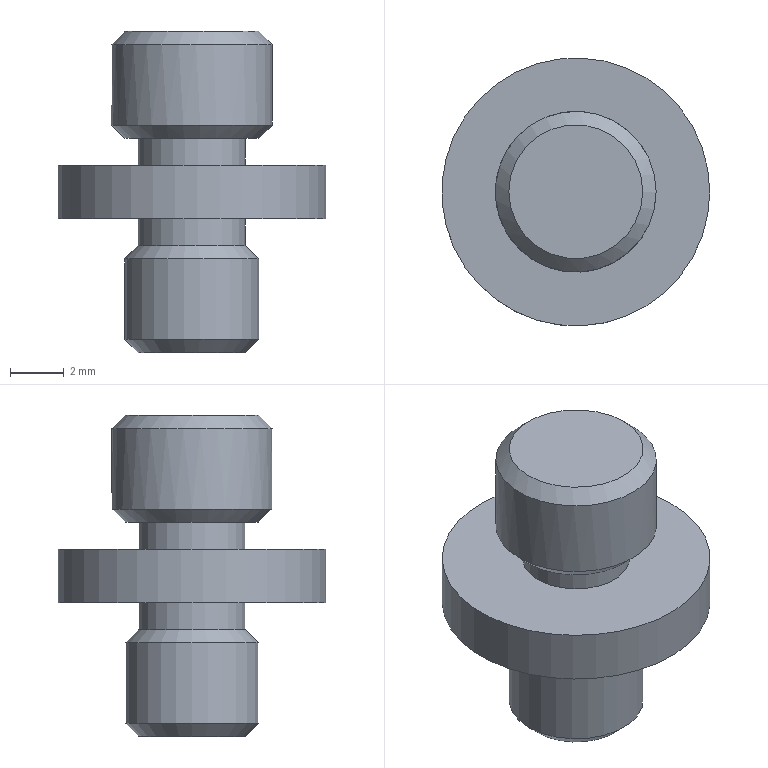Component | NX | DOWEL_PIN | 1 solid | 14 faces | box 10 x 10 x 12 mm | volume 366 mm3 | plane 5 | cylinder 5 | cone 4 | commonest cylinder face diameters 4 x2 5 x1 10 x1 6 x1
STEP:
#1=CARTESIAN_POINT('',(0.,0.,0.));
#2=DIRECTION('',(0.,0.,1.));
#3=DIRECTION('',(1.,0.,0.));
#4=AXIS2_PLACEMENT_3D('',#1,#2,#3);
#5=CARTESIAN_POINT('',(319.101,26.5,8.));
#6=VERTEX_POINT('',#5);
#7=CARTESIAN_POINT('',(321.101,26.5,8.));
#8=DIRECTION('',(0.,0.,-1.));
#9=DIRECTION('',(-1.,0.,0.));
#10=AXIS2_PLACEMENT_3D('',#7,#8,#9);
#11=CIRCLE('',#10,2.);
#12=CARTESIAN_POINT('',(321.101,26.5,8.));
#13=DIRECTION('',(0.,0.,-1.));
#14=DIRECTION('',(-1.,0.,0.));
#15=AXIS2_PLACEMENT_3D('',#12,#13,#14);
#16=PLANE('',#15);
#17=CARTESIAN_POINT('',(0.,0.));
#18=DIRECTION('',(1.,0.));
#19=AXIS2_PLACEMENT_2D('',#17,#18);
#20=CIRCLE('',#19,2.);
#21=(GEOMETRIC_REPRESENTATION_CONTEXT(2)PARAMETRIC_REPRESENTATION_CONTEXT()REPRESENTATION_CONTEXT('',''));
#22=DEFINITIONAL_REPRESENTATION('',(#20),#21);
#23=PCURVE('',#16,#22);
#24=CARTESIAN_POINT('',(321.101,26.5,8.5));
#25=DIRECTION('',(0.,0.,1.));
#26=DIRECTION('',(1.,0.,0.));
#27=AXIS2_PLACEMENT_3D('',#24,#25,#26);
#28=CONICAL_SURFACE('',#27,2.5,0.7854);
#29=CARTESIAN_POINT('',(9.425,-0.5));
#30=DIRECTION('',(-1.,0.));
#31=VECTOR('',#30,1.);
#32=LINE('',#29,#31);
#33=(GEOMETRIC_REPRESENTATION_CONTEXT(2)PARAMETRIC_REPRESENTATION_CONTEXT()REPRESENTATION_CONTEXT('',''));
#34=DEFINITIONAL_REPRESENTATION('',(#32),#33);
#35=PCURVE('',#28,#34);
#36=SURFACE_CURVE('',#11,(#23,#35),.PCURVE_S1.);
#37=EDGE_CURVE('',#6,#6,#36,.T.);
#38=ORIENTED_EDGE('',*,*,#37,.T.);
#39=EDGE_LOOP('',(#38));
#40=FACE_BOUND('',#39,.T.);
#41=ADVANCED_FACE('',(#40),#16,.T.);
#42=CARTESIAN_POINT('',(318.601,26.5,8.5));
#43=VERTEX_POINT('',#42);
#44=CARTESIAN_POINT('',(323.601,26.5,8.5));
#45=VERTEX_POINT('',#44);
#46=CARTESIAN_POINT('',(321.101,26.5,8.5));
#47=DIRECTION('',(0.,0.,1.));
#48=DIRECTION('',(-1.,0.,0.));
#49=AXIS2_PLACEMENT_3D('',#46,#47,#48);
#50=CIRCLE('',#49,2.5);
#51=CARTESIAN_POINT('',(321.101,26.5,8.));
#52=DIRECTION('',(0.,0.,1.));
#53=DIRECTION('',(1.,0.,0.));
#54=AXIS2_PLACEMENT_3D('',#51,#52,#53);
#55=CYLINDRICAL_SURFACE('',#54,2.5);
#56=CARTESIAN_POINT('',(3.142,0.5));
#57=DIRECTION('',(1.,0.));
#58=VECTOR('',#57,1.);
#59=LINE('',#56,#58);
#60=(GEOMETRIC_REPRESENTATION_CONTEXT(2)PARAMETRIC_REPRESENTATION_CONTEXT()REPRESENTATION_CONTEXT('',''));
#61=DEFINITIONAL_REPRESENTATION('',(#59),#60);
#62=PCURVE('',#55,#61);
#63=CARTESIAN_POINT('',(3.142,0.));
#64=DIRECTION('',(1.,0.));
#65=VECTOR('',#64,1.);
#66=LINE('',#63,#65);
#67=(GEOMETRIC_REPRESENTATION_CONTEXT(2)PARAMETRIC_REPRESENTATION_CONTEXT()REPRESENTATION_CONTEXT('',''));
#68=DEFINITIONAL_REPRESENTATION('',(#66),#67);
#69=PCURVE('',#28,#68);
#70=SURFACE_CURVE('',#50,(#62,#69),.PCURVE_S1.);
#71=EDGE_CURVE('',#43,#45,#70,.T.);
#72=ORIENTED_EDGE('',*,*,#71,.T.);
#73=CARTESIAN_POINT('',(323.601,26.5,11.5));
#74=VERTEX_POINT('',#73);
#75=CARTESIAN_POINT('',(323.601,26.5,8.5));
#76=CARTESIAN_POINT('',(323.601,26.5,11.5));
#77=B_SPLINE_CURVE_WITH_KNOTS('',1,(#75,#76),.UNSPECIFIED.,.F.,.F.,(2,2),(0.5,3.5),.PIECEWISE_BEZIER_KNOTS.);
#78=CARTESIAN_POINT('',(6.283,0.));
#79=DIRECTION('',(0.,1.));
#80=VECTOR('',#79,1.);
#81=LINE('',#78,#80);
#82=(GEOMETRIC_REPRESENTATION_CONTEXT(2)PARAMETRIC_REPRESENTATION_CONTEXT()REPRESENTATION_CONTEXT('',''));
#83=DEFINITIONAL_REPRESENTATION('',(#81),#82);
#84=PCURVE('',#55,#83);
#85=CARTESIAN_POINT('',(0.,0.));
#86=DIRECTION('',(0.,1.));
#87=VECTOR('',#86,1.);
#88=LINE('',#85,#87);
#89=(GEOMETRIC_REPRESENTATION_CONTEXT(2)PARAMETRIC_REPRESENTATION_CONTEXT()REPRESENTATION_CONTEXT('',''));
#90=DEFINITIONAL_REPRESENTATION('',(#88),#89);
#91=PCURVE('',#55,#90);
#92=SEAM_CURVE('',#77,(#84,#91),.PCURVE_S1.);
#93=EDGE_CURVE('',#45,#74,#92,.T.);
#94=ORIENTED_EDGE('',*,*,#93,.T.);
#95=CARTESIAN_POINT('',(321.101,26.5,11.5));
#96=DIRECTION('',(0.,0.,-1.));
#97=DIRECTION('',(1.,0.,0.));
#98=AXIS2_PLACEMENT_3D('',#95,#96,#97);
#99=CIRCLE('',#98,2.5);
#100=CARTESIAN_POINT('',(6.283,3.5));
#101=DIRECTION('',(-1.,0.));
#102=VECTOR('',#101,1.);
#103=LINE('',#100,#102);
#104=(GEOMETRIC_REPRESENTATION_CONTEXT(2)PARAMETRIC_REPRESENTATION_CONTEXT()REPRESENTATION_CONTEXT('',''));
#105=DEFINITIONAL_REPRESENTATION('',(#103),#104);
#106=PCURVE('',#55,#105);
#107=CARTESIAN_POINT('',(321.101,26.5,11.5));
#108=DIRECTION('',(0.,0.,-1.));
#109=DIRECTION('',(-1.,0.,0.));
#110=AXIS2_PLACEMENT_3D('',#107,#108,#109);
#111=CONICAL_SURFACE('',#110,2.5,0.7854);
#112=CARTESIAN_POINT('',(3.142,0.));
#113=DIRECTION('',(1.,0.));
#114=VECTOR('',#113,1.);
#115=LINE('',#112,#114);
#116=(GEOMETRIC_REPRESENTATION_CONTEXT(2)PARAMETRIC_REPRESENTATION_CONTEXT()REPRESENTATION_CONTEXT('',''));
#117=DEFINITIONAL_REPRESENTATION('',(#115),#116);
#118=PCURVE('',#111,#117);
#119=SURFACE_CURVE('',#99,(#106,#118),.PCURVE_S1.);
#120=EDGE_CURVE('',#74,#74,#119,.T.);
#121=ORIENTED_EDGE('',*,*,#120,.T.);
#122=ORIENTED_EDGE('',*,*,#93,.F.);
#123=CARTESIAN_POINT('',(321.101,26.5,8.5));
#124=DIRECTION('',(0.,0.,1.));
#125=DIRECTION('',(-1.,0.,0.));
#126=AXIS2_PLACEMENT_3D('',#123,#124,#125);
#127=CIRCLE('',#126,2.5);
#128=CARTESIAN_POINT('',(-3.142,0.5));
#129=DIRECTION('',(1.,0.));
#130=VECTOR('',#129,1.);
#131=LINE('',#128,#130);
#132=(GEOMETRIC_REPRESENTATION_CONTEXT(2)PARAMETRIC_REPRESENTATION_CONTEXT()REPRESENTATION_CONTEXT('',''));
#133=DEFINITIONAL_REPRESENTATION('',(#131),#132);
#134=PCURVE('',#55,#133);
#135=CARTESIAN_POINT('',(3.142,0.));
#136=DIRECTION('',(1.,0.));
#137=VECTOR('',#136,1.);
#138=LINE('',#135,#137);
#139=(GEOMETRIC_REPRESENTATION_CONTEXT(2)PARAMETRIC_REPRESENTATION_CONTEXT()REPRESENTATION_CONTEXT('',''));
#140=DEFINITIONAL_REPRESENTATION('',(#138),#139);
#141=PCURVE('',#28,#140);
#142=SURFACE_CURVE('',#127,(#134,#141),.PCURVE_S1.);
#143=EDGE_CURVE('',#45,#43,#142,.T.);
#144=ORIENTED_EDGE('',*,*,#143,.T.);
#145=EDGE_LOOP('',(#72,#94,#121,#122,#144));
#146=FACE_BOUND('',#145,.T.);
#147=ADVANCED_FACE('',(#146),#55,.T.);
#148=CARTESIAN_POINT('',(323.101,26.5,13.));
#149=VERTEX_POINT('',#148);
#150=CARTESIAN_POINT('',(321.101,26.5,13.));
#151=DIRECTION('',(0.,0.,-1.));
#152=DIRECTION('',(1.,0.,0.));
#153=AXIS2_PLACEMENT_3D('',#150,#151,#152);
#154=CIRCLE('',#153,2.);
#155=CARTESIAN_POINT('',(321.101,26.5,12.));
#156=DIRECTION('',(0.,0.,1.));
#157=DIRECTION('',(1.,0.,0.));
#158=AXIS2_PLACEMENT_3D('',#155,#156,#157);
#159=CYLINDRICAL_SURFACE('',#158,2.);
#160=CARTESIAN_POINT('',(6.283,1.));
#161=DIRECTION('',(-1.,0.));
#162=VECTOR('',#161,1.);
#163=LINE('',#160,#162);
#164=(GEOMETRIC_REPRESENTATION_CONTEXT(2)PARAMETRIC_REPRESENTATION_CONTEXT()REPRESENTATION_CONTEXT('',''));
#165=DEFINITIONAL_REPRESENTATION('',(#163),#164);
#166=PCURVE('',#159,#165);
#167=CARTESIAN_POINT('',(321.101,26.5,13.));
#168=DIRECTION('',(0.,0.,-1.));
#169=DIRECTION('',(-1.,0.,0.));
#170=AXIS2_PLACEMENT_3D('',#167,#168,#169);
#171=PLANE('',#170);
#172=CARTESIAN_POINT('',(0.,0.));
#173=DIRECTION('',(-1.,0.));
#174=AXIS2_PLACEMENT_2D('',#172,#173);
#175=CIRCLE('',#174,2.);
#176=(GEOMETRIC_REPRESENTATION_CONTEXT(2)PARAMETRIC_REPRESENTATION_CONTEXT()REPRESENTATION_CONTEXT('',''));
#177=DEFINITIONAL_REPRESENTATION('',(#175),#176);
#178=PCURVE('',#171,#177);
#179=SURFACE_CURVE('',#154,(#166,#178),.PCURVE_S1.);
#180=EDGE_CURVE('',#149,#149,#179,.T.);
#181=ORIENTED_EDGE('',*,*,#180,.T.);
#182=CARTESIAN_POINT('',(323.101,26.5,12.));
#183=VERTEX_POINT('',#182);
#184=CARTESIAN_POINT('',(323.101,26.5,12.));
#185=CARTESIAN_POINT('',(323.101,26.5,13.));
#186=B_SPLINE_CURVE_WITH_KNOTS('',1,(#184,#185),.UNSPECIFIED.,.F.,.F.,(2,2),(0.,1.),.PIECEWISE_BEZIER_KNOTS.);
#187=CARTESIAN_POINT('',(0.,0.));
#188=DIRECTION('',(0.,1.));
#189=VECTOR('',#188,1.);
#190=LINE('',#187,#189);
#191=(GEOMETRIC_REPRESENTATION_CONTEXT(2)PARAMETRIC_REPRESENTATION_CONTEXT()REPRESENTATION_CONTEXT('',''));
#192=DEFINITIONAL_REPRESENTATION('',(#190),#191);
#193=PCURVE('',#159,#192);
#194=CARTESIAN_POINT('',(6.283,0.));
#195=DIRECTION('',(0.,1.));
#196=VECTOR('',#195,1.);
#197=LINE('',#194,#196);
#198=(GEOMETRIC_REPRESENTATION_CONTEXT(2)PARAMETRIC_REPRESENTATION_CONTEXT()REPRESENTATION_CONTEXT('',''));
#199=DEFINITIONAL_REPRESENTATION('',(#197),#198);
#200=PCURVE('',#159,#199);
#201=SEAM_CURVE('',#186,(#193,#200),.PCURVE_S1.);
#202=EDGE_CURVE('',#183,#149,#201,.T.);
#203=ORIENTED_EDGE('',*,*,#202,.F.);
#204=CARTESIAN_POINT('',(321.101,26.5,12.));
#205=DIRECTION('',(0.,0.,1.));
#206=DIRECTION('',(1.,0.,0.));
#207=AXIS2_PLACEMENT_3D('',#204,#205,#206);
#208=CIRCLE('',#207,2.);
#209=CARTESIAN_POINT('',(0.,0.));
#210=DIRECTION('',(1.,0.));
#211=VECTOR('',#210,1.);
#212=LINE('',#209,#211);
#213=(GEOMETRIC_REPRESENTATION_CONTEXT(2)PARAMETRIC_REPRESENTATION_CONTEXT()REPRESENTATION_CONTEXT('',''));
#214=DEFINITIONAL_REPRESENTATION('',(#212),#213);
#215=PCURVE('',#159,#214);
#216=CARTESIAN_POINT('',(9.425,-0.5));
#217=DIRECTION('',(-1.,0.));
#218=VECTOR('',#217,1.);
#219=LINE('',#216,#218);
#220=(GEOMETRIC_REPRESENTATION_CONTEXT(2)PARAMETRIC_REPRESENTATION_CONTEXT()REPRESENTATION_CONTEXT('',''));
#221=DEFINITIONAL_REPRESENTATION('',(#219),#220);
#222=PCURVE('',#111,#221);
#223=SURFACE_CURVE('',#208,(#215,#222),.PCURVE_S1.);
#224=EDGE_CURVE('',#183,#183,#223,.T.);
#225=ORIENTED_EDGE('',*,*,#224,.T.);
#226=ORIENTED_EDGE('',*,*,#202,.T.);
#227=EDGE_LOOP('',(#181,#203,#225,#226));
#228=FACE_BOUND('',#227,.T.);
#229=ADVANCED_FACE('',(#228),#159,.T.);
#230=CARTESIAN_POINT('',(323.101,26.5,15.));
#231=VERTEX_POINT('',#230);
#232=CARTESIAN_POINT('',(321.101,26.5,15.));
#233=DIRECTION('',(0.,0.,1.));
#234=DIRECTION('',(1.,0.,0.));
#235=AXIS2_PLACEMENT_3D('',#232,#233,#234);
#236=CIRCLE('',#235,2.);
#237=CARTESIAN_POINT('',(321.101,26.5,15.));
#238=DIRECTION('',(0.,0.,1.));
#239=DIRECTION('',(1.,0.,0.));
#240=AXIS2_PLACEMENT_3D('',#237,#238,#239);
#241=PLANE('',#240);
#242=CARTESIAN_POINT('',(0.,0.));
#243=DIRECTION('',(1.,0.));
#244=AXIS2_PLACEMENT_2D('',#242,#243);
#245=CIRCLE('',#244,2.);
#246=(GEOMETRIC_REPRESENTATION_CONTEXT(2)PARAMETRIC_REPRESENTATION_CONTEXT()REPRESENTATION_CONTEXT('',''));
#247=DEFINITIONAL_REPRESENTATION('',(#245),#246);
#248=PCURVE('',#241,#247);
#249=CARTESIAN_POINT('',(321.101,26.5,15.));
#250=DIRECTION('',(0.,0.,1.));
#251=DIRECTION('',(1.,0.,0.));
#252=AXIS2_PLACEMENT_3D('',#249,#250,#251);
#253=CYLINDRICAL_SURFACE('',#252,2.);
#254=CARTESIAN_POINT('',(0.,0.));
#255=DIRECTION('',(1.,0.));
#256=VECTOR('',#255,1.);
#257=LINE('',#254,#256);
#258=(GEOMETRIC_REPRESENTATION_CONTEXT(2)PARAMETRIC_REPRESENTATION_CONTEXT()REPRESENTATION_CONTEXT('',''));
#259=DEFINITIONAL_REPRESENTATION('',(#257),#258);
#260=PCURVE('',#253,#259);
#261=SURFACE_CURVE('',#236,(#248,#260),.PCURVE_S1.);
#262=EDGE_CURVE('',#231,#231,#261,.T.);
#263=ORIENTED_EDGE('',*,*,#262,.F.);
#264=EDGE_LOOP('',(#263));
#265=FACE_BOUND('',#264,.T.);
#266=CARTESIAN_POINT('',(326.101,26.5,15.));
#267=VERTEX_POINT('',#266);
#268=CARTESIAN_POINT('',(321.101,26.5,15.));
#269=DIRECTION('',(0.,0.,-1.));
#270=DIRECTION('',(1.,0.,0.));
#271=AXIS2_PLACEMENT_3D('',#268,#269,#270);
#272=CIRCLE('',#271,5.);
#273=CARTESIAN_POINT('',(5.,0.));
#274=CARTESIAN_POINT('',(5.,-8.66));
#275=CARTESIAN_POINT('',(-2.5,-4.33));
#276=CARTESIAN_POINT('',(-10.,-0.));
#277=CARTESIAN_POINT('',(-2.5,4.33));
#278=CARTESIAN_POINT('',(5.,8.66));
#279=CARTESIAN_POINT('',(5.,0.));
#280=(BOUNDED_CURVE()B_SPLINE_CURVE(2,(#273,#274,#275,#276,#277,#278,#279),.UNSPECIFIED.,.T.,.F.)B_SPLINE_CURVE_WITH_KNOTS((1,2,2,2,2,1),(-2.094,0.,2.094,4.189,6.283,8.378),.UNSPECIFIED.)CURVE()GEOMETRIC_REPRESENTATION_ITEM()RATIONAL_B_SPLINE_CURVE((1.,0.5,1.,0.5,1.,0.5,1.))REPRESENTATION_ITEM(''));
#281=(GEOMETRIC_REPRESENTATION_CONTEXT(2)PARAMETRIC_REPRESENTATION_CONTEXT()REPRESENTATION_CONTEXT('',''));
#282=DEFINITIONAL_REPRESENTATION('',(#280),#281);
#283=PCURVE('',#241,#282);
#284=CARTESIAN_POINT('',(321.101,26.5,13.));
#285=DIRECTION('',(0.,0.,1.));
#286=DIRECTION('',(1.,0.,0.));
#287=AXIS2_PLACEMENT_3D('',#284,#285,#286);
#288=CYLINDRICAL_SURFACE('',#287,5.);
#289=CARTESIAN_POINT('',(6.283,2.));
#290=DIRECTION('',(-1.,0.));
#291=VECTOR('',#290,1.);
#292=LINE('',#289,#291);
#293=(GEOMETRIC_REPRESENTATION_CONTEXT(2)PARAMETRIC_REPRESENTATION_CONTEXT()REPRESENTATION_CONTEXT('',''));
#294=DEFINITIONAL_REPRESENTATION('',(#292),#293);
#295=PCURVE('',#288,#294);
#296=SURFACE_CURVE('',#272,(#283,#295),.PCURVE_S1.);
#297=EDGE_CURVE('',#267,#267,#296,.T.);
#298=ORIENTED_EDGE('',*,*,#297,.F.);
#299=EDGE_LOOP('',(#298));
#300=FACE_BOUND('',#299,.T.);
#301=ADVANCED_FACE('',(#265,#300),#241,.T.);
#302=ORIENTED_EDGE('',*,*,#180,.F.);
#303=EDGE_LOOP('',(#302));
#304=FACE_BOUND('',#303,.T.);
#305=CARTESIAN_POINT('',(326.101,26.5,13.));
#306=VERTEX_POINT('',#305);
#307=CARTESIAN_POINT('',(321.101,26.5,13.));
#308=DIRECTION('',(0.,0.,1.));
#309=DIRECTION('',(1.,0.,0.));
#310=AXIS2_PLACEMENT_3D('',#307,#308,#309);
#311=CIRCLE('',#310,5.);
#312=CARTESIAN_POINT('',(-5.,0.));
#313=CARTESIAN_POINT('',(-5.,8.66));
#314=CARTESIAN_POINT('',(2.5,4.33));
#315=CARTESIAN_POINT('',(10.,0.));
#316=CARTESIAN_POINT('',(2.5,-4.33));
#317=CARTESIAN_POINT('',(-5.,-8.66));
#318=CARTESIAN_POINT('',(-5.,0.));
#319=(BOUNDED_CURVE()B_SPLINE_CURVE(2,(#312,#313,#314,#315,#316,#317,#318),.UNSPECIFIED.,.T.,.F.)B_SPLINE_CURVE_WITH_KNOTS((1,2,2,2,2,1),(-2.094,0.,2.094,4.189,6.283,8.378),.UNSPECIFIED.)CURVE()GEOMETRIC_REPRESENTATION_ITEM()RATIONAL_B_SPLINE_CURVE((1.,0.5,1.,0.5,1.,0.5,1.))REPRESENTATION_ITEM(''));
#320=(GEOMETRIC_REPRESENTATION_CONTEXT(2)PARAMETRIC_REPRESENTATION_CONTEXT()REPRESENTATION_CONTEXT('',''));
#321=DEFINITIONAL_REPRESENTATION('',(#319),#320);
#322=PCURVE('',#171,#321);
#323=CARTESIAN_POINT('',(0.,0.));
#324=DIRECTION('',(1.,0.));
#325=VECTOR('',#324,1.);
#326=LINE('',#323,#325);
#327=(GEOMETRIC_REPRESENTATION_CONTEXT(2)PARAMETRIC_REPRESENTATION_CONTEXT()REPRESENTATION_CONTEXT('',''));
#328=DEFINITIONAL_REPRESENTATION('',(#326),#327);
#329=PCURVE('',#288,#328);
#330=SURFACE_CURVE('',#311,(#322,#329),.PCURVE_S1.);
#331=EDGE_CURVE('',#306,#306,#330,.T.);
#332=ORIENTED_EDGE('',*,*,#331,.F.);
#333=EDGE_LOOP('',(#332));
#334=FACE_BOUND('',#333,.T.);
#335=ADVANCED_FACE('',(#304,#334),#171,.T.);
#336=ORIENTED_EDGE('',*,*,#297,.T.);
#337=CARTESIAN_POINT('',(326.101,26.5,13.));
#338=CARTESIAN_POINT('',(326.101,26.5,15.));
#339=B_SPLINE_CURVE_WITH_KNOTS('',1,(#337,#338),.UNSPECIFIED.,.F.,.F.,(2,2),(0.,2.),.PIECEWISE_BEZIER_KNOTS.);
#340=CARTESIAN_POINT('',(0.,0.));
#341=DIRECTION('',(0.,1.));
#342=VECTOR('',#341,1.);
#343=LINE('',#340,#342);
#344=(GEOMETRIC_REPRESENTATION_CONTEXT(2)PARAMETRIC_REPRESENTATION_CONTEXT()REPRESENTATION_CONTEXT('',''));
#345=DEFINITIONAL_REPRESENTATION('',(#343),#344);
#346=PCURVE('',#288,#345);
#347=CARTESIAN_POINT('',(6.283,0.));
#348=DIRECTION('',(0.,1.));
#349=VECTOR('',#348,1.);
#350=LINE('',#347,#349);
#351=(GEOMETRIC_REPRESENTATION_CONTEXT(2)PARAMETRIC_REPRESENTATION_CONTEXT()REPRESENTATION_CONTEXT('',''));
#352=DEFINITIONAL_REPRESENTATION('',(#350),#351);
#353=PCURVE('',#288,#352);
#354=SEAM_CURVE('',#339,(#346,#353),.PCURVE_S1.);
#355=EDGE_CURVE('',#306,#267,#354,.T.);
#356=ORIENTED_EDGE('',*,*,#355,.F.);
#357=ORIENTED_EDGE('',*,*,#331,.T.);
#358=ORIENTED_EDGE('',*,*,#355,.T.);
#359=EDGE_LOOP('',(#336,#356,#357,#358));
#360=FACE_BOUND('',#359,.T.);
#361=ADVANCED_FACE('',(#360),#288,.T.);
#362=CARTESIAN_POINT('',(323.101,26.5,16.));
#363=VERTEX_POINT('',#362);
#364=CARTESIAN_POINT('',(321.101,26.5,16.));
#365=DIRECTION('',(0.,0.,-1.));
#366=DIRECTION('',(1.,0.,0.));
#367=AXIS2_PLACEMENT_3D('',#364,#365,#366);
#368=CIRCLE('',#367,2.);
#369=CARTESIAN_POINT('',(6.283,1.));
#370=DIRECTION('',(-1.,0.));
#371=VECTOR('',#370,1.);
#372=LINE('',#369,#371);
#373=(GEOMETRIC_REPRESENTATION_CONTEXT(2)PARAMETRIC_REPRESENTATION_CONTEXT()REPRESENTATION_CONTEXT('',''));
#374=DEFINITIONAL_REPRESENTATION('',(#372),#373);
#375=PCURVE('',#253,#374);
#376=CARTESIAN_POINT('',(321.101,26.5,16.));
#377=DIRECTION('',(0.,0.,-1.));
#378=DIRECTION('',(-1.,0.,0.));
#379=AXIS2_PLACEMENT_3D('',#376,#377,#378);
#380=PLANE('',#379);
#381=CARTESIAN_POINT('',(0.,0.));
#382=DIRECTION('',(-1.,0.));
#383=AXIS2_PLACEMENT_2D('',#381,#382);
#384=CIRCLE('',#383,2.);
#385=(GEOMETRIC_REPRESENTATION_CONTEXT(2)PARAMETRIC_REPRESENTATION_CONTEXT()REPRESENTATION_CONTEXT('',''));
#386=DEFINITIONAL_REPRESENTATION('',(#384),#385);
#387=PCURVE('',#380,#386);
#388=SURFACE_CURVE('',#368,(#375,#387),.PCURVE_S1.);
#389=EDGE_CURVE('',#363,#363,#388,.T.);
#390=ORIENTED_EDGE('',*,*,#389,.T.);
#391=CARTESIAN_POINT('',(323.101,26.5,15.));
#392=CARTESIAN_POINT('',(323.101,26.5,16.));
#393=B_SPLINE_CURVE_WITH_KNOTS('',1,(#391,#392),.UNSPECIFIED.,.F.,.F.,(2,2),(0.,1.),.PIECEWISE_BEZIER_KNOTS.);
#394=CARTESIAN_POINT('',(0.,0.));
#395=DIRECTION('',(0.,1.));
#396=VECTOR('',#395,1.);
#397=LINE('',#394,#396);
#398=(GEOMETRIC_REPRESENTATION_CONTEXT(2)PARAMETRIC_REPRESENTATION_CONTEXT()REPRESENTATION_CONTEXT('',''));
#399=DEFINITIONAL_REPRESENTATION('',(#397),#398);
#400=PCURVE('',#253,#399);
#401=CARTESIAN_POINT('',(6.283,0.));
#402=DIRECTION('',(0.,1.));
#403=VECTOR('',#402,1.);
#404=LINE('',#401,#403);
#405=(GEOMETRIC_REPRESENTATION_CONTEXT(2)PARAMETRIC_REPRESENTATION_CONTEXT()REPRESENTATION_CONTEXT('',''));
#406=DEFINITIONAL_REPRESENTATION('',(#404),#405);
#407=PCURVE('',#253,#406);
#408=SEAM_CURVE('',#393,(#400,#407),.PCURVE_S1.);
#409=EDGE_CURVE('',#231,#363,#408,.T.);
#410=ORIENTED_EDGE('',*,*,#409,.F.);
#411=ORIENTED_EDGE('',*,*,#262,.T.);
#412=ORIENTED_EDGE('',*,*,#409,.T.);
#413=EDGE_LOOP('',(#390,#410,#411,#412));
#414=FACE_BOUND('',#413,.T.);
#415=ADVANCED_FACE('',(#414),#253,.T.);
#416=CARTESIAN_POINT('',(323.601,26.5,20.));
#417=VERTEX_POINT('',#416);
#418=CARTESIAN_POINT('',(321.101,26.5,20.));
#419=DIRECTION('',(0.,0.,1.));
#420=DIRECTION('',(1.,0.,0.));
#421=AXIS2_PLACEMENT_3D('',#418,#419,#420);
#422=CIRCLE('',#421,2.5);
#423=CARTESIAN_POINT('',(321.101,26.5,20.));
#424=DIRECTION('',(0.,0.,1.));
#425=DIRECTION('',(1.,0.,0.));
#426=AXIS2_PLACEMENT_3D('',#423,#424,#425);
#427=PLANE('',#426);
#428=CARTESIAN_POINT('',(0.,0.));
#429=DIRECTION('',(1.,0.));
#430=AXIS2_PLACEMENT_2D('',#428,#429);
#431=CIRCLE('',#430,2.5);
#432=(GEOMETRIC_REPRESENTATION_CONTEXT(2)PARAMETRIC_REPRESENTATION_CONTEXT()REPRESENTATION_CONTEXT('',''));
#433=DEFINITIONAL_REPRESENTATION('',(#431),#432);
#434=PCURVE('',#427,#433);
#435=CARTESIAN_POINT('',(321.101,26.5,19.5));
#436=DIRECTION('',(0.,0.,-1.));
#437=DIRECTION('',(-1.,0.,0.));
#438=AXIS2_PLACEMENT_3D('',#435,#436,#437);
#439=CONICAL_SURFACE('',#438,3.,0.7854);
#440=CARTESIAN_POINT('',(9.425,-0.5));
#441=DIRECTION('',(-1.,0.));
#442=VECTOR('',#441,1.);
#443=LINE('',#440,#442);
#444=(GEOMETRIC_REPRESENTATION_CONTEXT(2)PARAMETRIC_REPRESENTATION_CONTEXT()REPRESENTATION_CONTEXT('',''));
#445=DEFINITIONAL_REPRESENTATION('',(#443),#444);
#446=PCURVE('',#439,#445);
#447=SURFACE_CURVE('',#422,(#434,#446),.PCURVE_S1.);
#448=EDGE_CURVE('',#417,#417,#447,.T.);
#449=ORIENTED_EDGE('',*,*,#448,.T.);
#450=EDGE_LOOP('',(#449));
#451=FACE_BOUND('',#450,.T.);
#452=ADVANCED_FACE('',(#451),#427,.T.);
#453=CARTESIAN_POINT('',(318.601,26.5,16.));
#454=VERTEX_POINT('',#453);
#455=CARTESIAN_POINT('',(321.101,26.5,16.));
#456=DIRECTION('',(0.,0.,-1.));
#457=DIRECTION('',(-1.,0.,0.));
#458=AXIS2_PLACEMENT_3D('',#455,#456,#457);
#459=CIRCLE('',#458,2.5);
#460=CARTESIAN_POINT('',(0.,0.));
#461=DIRECTION('',(1.,0.));
#462=AXIS2_PLACEMENT_2D('',#460,#461);
#463=CIRCLE('',#462,2.5);
#464=(GEOMETRIC_REPRESENTATION_CONTEXT(2)PARAMETRIC_REPRESENTATION_CONTEXT()REPRESENTATION_CONTEXT('',''));
#465=DEFINITIONAL_REPRESENTATION('',(#463),#464);
#466=PCURVE('',#380,#465);
#467=CARTESIAN_POINT('',(321.101,26.5,16.5));
#468=DIRECTION('',(0.,0.,1.));
#469=DIRECTION('',(1.,0.,0.));
#470=AXIS2_PLACEMENT_3D('',#467,#468,#469);
#471=CONICAL_SURFACE('',#470,3.,0.7854);
#472=CARTESIAN_POINT('',(9.425,-0.5));
#473=DIRECTION('',(-1.,0.));
#474=VECTOR('',#473,1.);
#475=LINE('',#472,#474);
#476=(GEOMETRIC_REPRESENTATION_CONTEXT(2)PARAMETRIC_REPRESENTATION_CONTEXT()REPRESENTATION_CONTEXT('',''));
#477=DEFINITIONAL_REPRESENTATION('',(#475),#476);
#478=PCURVE('',#471,#477);
#479=SURFACE_CURVE('',#459,(#466,#478),.PCURVE_S1.);
#480=EDGE_CURVE('',#454,#454,#479,.T.);
#481=ORIENTED_EDGE('',*,*,#480,.T.);
#482=EDGE_LOOP('',(#481));
#483=FACE_BOUND('',#482,.T.);
#484=ORIENTED_EDGE('',*,*,#389,.F.);
#485=EDGE_LOOP('',(#484));
#486=FACE_BOUND('',#485,.T.);
#487=ADVANCED_FACE('',(#483,#486),#380,.T.);
#488=CARTESIAN_POINT('',(318.101,26.5,16.5));
#489=VERTEX_POINT('',#488);
#490=CARTESIAN_POINT('',(324.101,26.5,16.5));
#491=VERTEX_POINT('',#490);
#492=CARTESIAN_POINT('',(321.101,26.5,16.5));
#493=DIRECTION('',(0.,0.,1.));
#494=DIRECTION('',(-1.,0.,0.));
#495=AXIS2_PLACEMENT_3D('',#492,#493,#494);
#496=CIRCLE('',#495,3.);
#497=CARTESIAN_POINT('',(321.101,26.5,16.));
#498=DIRECTION('',(0.,0.,1.));
#499=DIRECTION('',(1.,0.,0.));
#500=AXIS2_PLACEMENT_3D('',#497,#498,#499);
#501=CYLINDRICAL_SURFACE('',#500,3.);
#502=CARTESIAN_POINT('',(3.142,0.5));
#503=DIRECTION('',(1.,0.));
#504=VECTOR('',#503,1.);
#505=LINE('',#502,#504);
#506=(GEOMETRIC_REPRESENTATION_CONTEXT(2)PARAMETRIC_REPRESENTATION_CONTEXT()REPRESENTATION_CONTEXT('',''));
#507=DEFINITIONAL_REPRESENTATION('',(#505),#506);
#508=PCURVE('',#501,#507);
#509=CARTESIAN_POINT('',(3.142,0.));
#510=DIRECTION('',(1.,0.));
#511=VECTOR('',#510,1.);
#512=LINE('',#509,#511);
#513=(GEOMETRIC_REPRESENTATION_CONTEXT(2)PARAMETRIC_REPRESENTATION_CONTEXT()REPRESENTATION_CONTEXT('',''));
#514=DEFINITIONAL_REPRESENTATION('',(#512),#513);
#515=PCURVE('',#471,#514);
#516=SURFACE_CURVE('',#496,(#508,#515),.PCURVE_S1.);
#517=EDGE_CURVE('',#489,#491,#516,.T.);
#518=ORIENTED_EDGE('',*,*,#517,.T.);
#519=CARTESIAN_POINT('',(324.101,26.5,19.5));
#520=VERTEX_POINT('',#519);
#521=CARTESIAN_POINT('',(324.101,26.5,16.5));
#522=CARTESIAN_POINT('',(324.101,26.5,19.5));
#523=B_SPLINE_CURVE_WITH_KNOTS('',1,(#521,#522),.UNSPECIFIED.,.F.,.F.,(2,2),(0.5,3.5),.PIECEWISE_BEZIER_KNOTS.);
#524=CARTESIAN_POINT('',(6.283,0.));
#525=DIRECTION('',(0.,1.));
#526=VECTOR('',#525,1.);
#527=LINE('',#524,#526);
#528=(GEOMETRIC_REPRESENTATION_CONTEXT(2)PARAMETRIC_REPRESENTATION_CONTEXT()REPRESENTATION_CONTEXT('',''));
#529=DEFINITIONAL_REPRESENTATION('',(#527),#528);
#530=PCURVE('',#501,#529);
#531=CARTESIAN_POINT('',(0.,0.));
#532=DIRECTION('',(0.,1.));
#533=VECTOR('',#532,1.);
#534=LINE('',#531,#533);
#535=(GEOMETRIC_REPRESENTATION_CONTEXT(2)PARAMETRIC_REPRESENTATION_CONTEXT()REPRESENTATION_CONTEXT('',''));
#536=DEFINITIONAL_REPRESENTATION('',(#534),#535);
#537=PCURVE('',#501,#536);
#538=SEAM_CURVE('',#523,(#530,#537),.PCURVE_S1.);
#539=EDGE_CURVE('',#491,#520,#538,.T.);
#540=ORIENTED_EDGE('',*,*,#539,.T.);
#541=CARTESIAN_POINT('',(321.101,26.5,19.5));
#542=DIRECTION('',(0.,0.,-1.));
#543=DIRECTION('',(1.,0.,0.));
#544=AXIS2_PLACEMENT_3D('',#541,#542,#543);
#545=CIRCLE('',#544,3.);
#546=CARTESIAN_POINT('',(6.283,3.5));
#547=DIRECTION('',(-1.,0.));
#548=VECTOR('',#547,1.);
#549=LINE('',#546,#548);
#550=(GEOMETRIC_REPRESENTATION_CONTEXT(2)PARAMETRIC_REPRESENTATION_CONTEXT()REPRESENTATION_CONTEXT('',''));
#551=DEFINITIONAL_REPRESENTATION('',(#549),#550);
#552=PCURVE('',#501,#551);
#553=CARTESIAN_POINT('',(3.142,0.));
#554=DIRECTION('',(1.,0.));
#555=VECTOR('',#554,1.);
#556=LINE('',#553,#555);
#557=(GEOMETRIC_REPRESENTATION_CONTEXT(2)PARAMETRIC_REPRESENTATION_CONTEXT()REPRESENTATION_CONTEXT('',''));
#558=DEFINITIONAL_REPRESENTATION('',(#556),#557);
#559=PCURVE('',#439,#558);
#560=SURFACE_CURVE('',#545,(#552,#559),.PCURVE_S1.);
#561=EDGE_CURVE('',#520,#520,#560,.T.);
#562=ORIENTED_EDGE('',*,*,#561,.T.);
#563=ORIENTED_EDGE('',*,*,#539,.F.);
#564=CARTESIAN_POINT('',(321.101,26.5,16.5));
#565=DIRECTION('',(0.,0.,1.));
#566=DIRECTION('',(-1.,0.,0.));
#567=AXIS2_PLACEMENT_3D('',#564,#565,#566);
#568=CIRCLE('',#567,3.);
#569=CARTESIAN_POINT('',(-3.142,0.5));
#570=DIRECTION('',(1.,0.));
#571=VECTOR('',#570,1.);
#572=LINE('',#569,#571);
#573=(GEOMETRIC_REPRESENTATION_CONTEXT(2)PARAMETRIC_REPRESENTATION_CONTEXT()REPRESENTATION_CONTEXT('',''));
#574=DEFINITIONAL_REPRESENTATION('',(#572),#573);
#575=PCURVE('',#501,#574);
#576=CARTESIAN_POINT('',(3.142,0.));
#577=DIRECTION('',(1.,0.));
#578=VECTOR('',#577,1.);
#579=LINE('',#576,#578);
#580=(GEOMETRIC_REPRESENTATION_CONTEXT(2)PARAMETRIC_REPRESENTATION_CONTEXT()REPRESENTATION_CONTEXT('',''));
#581=DEFINITIONAL_REPRESENTATION('',(#579),#580);
#582=PCURVE('',#471,#581);
#583=SURFACE_CURVE('',#568,(#575,#582),.PCURVE_S1.);
#584=EDGE_CURVE('',#491,#489,#583,.T.);
#585=ORIENTED_EDGE('',*,*,#584,.T.);
#586=EDGE_LOOP('',(#518,#540,#562,#563,#585));
#587=FACE_BOUND('',#586,.T.);
#588=ADVANCED_FACE('',(#587),#501,.T.);
#589=ORIENTED_EDGE('',*,*,#37,.F.);
#590=CARTESIAN_POINT('',(319.101,26.5,8.));
#591=CARTESIAN_POINT('',(318.601,26.5,8.5));
#592=B_SPLINE_CURVE_WITH_KNOTS('',1,(#590,#591),.UNSPECIFIED.,.F.,.F.,(2,2),(-0.7071,0.),.PIECEWISE_BEZIER_KNOTS.);
#593=CARTESIAN_POINT('',(9.425,0.));
#594=DIRECTION('',(0.,1.));
#595=VECTOR('',#594,1.);
#596=LINE('',#593,#595);
#597=(GEOMETRIC_REPRESENTATION_CONTEXT(2)PARAMETRIC_REPRESENTATION_CONTEXT()REPRESENTATION_CONTEXT('',''));
#598=DEFINITIONAL_REPRESENTATION('',(#596),#597);
#599=PCURVE('',#28,#598);
#600=CARTESIAN_POINT('',(3.142,0.));
#601=DIRECTION('',(0.,1.));
#602=VECTOR('',#601,1.);
#603=LINE('',#600,#602);
#604=(GEOMETRIC_REPRESENTATION_CONTEXT(2)PARAMETRIC_REPRESENTATION_CONTEXT()REPRESENTATION_CONTEXT('',''));
#605=DEFINITIONAL_REPRESENTATION('',(#603),#604);
#606=PCURVE('',#28,#605);
#607=SEAM_CURVE('',#592,(#599,#606),.PCURVE_S1.);
#608=EDGE_CURVE('',#6,#43,#607,.T.);
#609=ORIENTED_EDGE('',*,*,#608,.T.);
#610=ORIENTED_EDGE('',*,*,#143,.F.);
#611=ORIENTED_EDGE('',*,*,#71,.F.);
#612=ORIENTED_EDGE('',*,*,#608,.F.);
#613=EDGE_LOOP('',(#589,#609,#610,#611,#612));
#614=FACE_BOUND('',#613,.T.);
#615=ADVANCED_FACE('',(#614),#28,.T.);
#616=ORIENTED_EDGE('',*,*,#224,.F.);
#617=CARTESIAN_POINT('',(323.101,26.5,12.));
#618=CARTESIAN_POINT('',(323.601,26.5,11.5));
#619=B_SPLINE_CURVE_WITH_KNOTS('',1,(#617,#618),.UNSPECIFIED.,.F.,.F.,(2,2),(-0.7071,0.),.PIECEWISE_BEZIER_KNOTS.);
#620=CARTESIAN_POINT('',(9.425,0.));
#621=DIRECTION('',(0.,1.));
#622=VECTOR('',#621,1.);
#623=LINE('',#620,#622);
#624=(GEOMETRIC_REPRESENTATION_CONTEXT(2)PARAMETRIC_REPRESENTATION_CONTEXT()REPRESENTATION_CONTEXT('',''));
#625=DEFINITIONAL_REPRESENTATION('',(#623),#624);
#626=PCURVE('',#111,#625);
#627=CARTESIAN_POINT('',(3.142,0.));
#628=DIRECTION('',(0.,1.));
#629=VECTOR('',#628,1.);
#630=LINE('',#627,#629);
#631=(GEOMETRIC_REPRESENTATION_CONTEXT(2)PARAMETRIC_REPRESENTATION_CONTEXT()REPRESENTATION_CONTEXT('',''));
#632=DEFINITIONAL_REPRESENTATION('',(#630),#631);
#633=PCURVE('',#111,#632);
#634=SEAM_CURVE('',#619,(#626,#633),.PCURVE_S1.);
#635=EDGE_CURVE('',#183,#74,#634,.T.);
#636=ORIENTED_EDGE('',*,*,#635,.T.);
#637=ORIENTED_EDGE('',*,*,#120,.F.);
#638=ORIENTED_EDGE('',*,*,#635,.F.);
#639=EDGE_LOOP('',(#616,#636,#637,#638));
#640=FACE_BOUND('',#639,.T.);
#641=ADVANCED_FACE('',(#640),#111,.T.);
#642=ORIENTED_EDGE('',*,*,#480,.F.);
#643=CARTESIAN_POINT('',(318.601,26.5,16.));
#644=CARTESIAN_POINT('',(318.101,26.5,16.5));
#645=B_SPLINE_CURVE_WITH_KNOTS('',1,(#643,#644),.UNSPECIFIED.,.F.,.F.,(2,2),(-0.7071,0.),.PIECEWISE_BEZIER_KNOTS.);
#646=CARTESIAN_POINT('',(9.425,0.));
#647=DIRECTION('',(0.,1.));
#648=VECTOR('',#647,1.);
#649=LINE('',#646,#648);
#650=(GEOMETRIC_REPRESENTATION_CONTEXT(2)PARAMETRIC_REPRESENTATION_CONTEXT()REPRESENTATION_CONTEXT('',''));
#651=DEFINITIONAL_REPRESENTATION('',(#649),#650);
#652=PCURVE('',#471,#651);
#653=CARTESIAN_POINT('',(3.142,0.));
#654=DIRECTION('',(0.,1.));
#655=VECTOR('',#654,1.);
#656=LINE('',#653,#655);
#657=(GEOMETRIC_REPRESENTATION_CONTEXT(2)PARAMETRIC_REPRESENTATION_CONTEXT()REPRESENTATION_CONTEXT('',''));
#658=DEFINITIONAL_REPRESENTATION('',(#656),#657);
#659=PCURVE('',#471,#658);
#660=SEAM_CURVE('',#645,(#652,#659),.PCURVE_S1.);
#661=EDGE_CURVE('',#454,#489,#660,.T.);
#662=ORIENTED_EDGE('',*,*,#661,.T.);
#663=ORIENTED_EDGE('',*,*,#584,.F.);
#664=ORIENTED_EDGE('',*,*,#517,.F.);
#665=ORIENTED_EDGE('',*,*,#661,.F.);
#666=EDGE_LOOP('',(#642,#662,#663,#664,#665));
#667=FACE_BOUND('',#666,.T.);
#668=ADVANCED_FACE('',(#667),#471,.T.);
#669=ORIENTED_EDGE('',*,*,#448,.F.);
#670=CARTESIAN_POINT('',(323.601,26.5,20.));
#671=CARTESIAN_POINT('',(324.101,26.5,19.5));
#672=B_SPLINE_CURVE_WITH_KNOTS('',1,(#670,#671),.UNSPECIFIED.,.F.,.F.,(2,2),(-0.7071,0.),.PIECEWISE_BEZIER_KNOTS.);
#673=CARTESIAN_POINT('',(9.425,0.));
#674=DIRECTION('',(0.,1.));
#675=VECTOR('',#674,1.);
#676=LINE('',#673,#675);
#677=(GEOMETRIC_REPRESENTATION_CONTEXT(2)PARAMETRIC_REPRESENTATION_CONTEXT()REPRESENTATION_CONTEXT('',''));
#678=DEFINITIONAL_REPRESENTATION('',(#676),#677);
#679=PCURVE('',#439,#678);
#680=CARTESIAN_POINT('',(3.142,0.));
#681=DIRECTION('',(0.,1.));
#682=VECTOR('',#681,1.);
#683=LINE('',#680,#682);
#684=(GEOMETRIC_REPRESENTATION_CONTEXT(2)PARAMETRIC_REPRESENTATION_CONTEXT()REPRESENTATION_CONTEXT('',''));
#685=DEFINITIONAL_REPRESENTATION('',(#683),#684);
#686=PCURVE('',#439,#685);
#687=SEAM_CURVE('',#672,(#679,#686),.PCURVE_S1.);
#688=EDGE_CURVE('',#417,#520,#687,.T.);
#689=ORIENTED_EDGE('',*,*,#688,.T.);
#690=ORIENTED_EDGE('',*,*,#561,.F.);
#691=ORIENTED_EDGE('',*,*,#688,.F.);
#692=EDGE_LOOP('',(#669,#689,#690,#691));
#693=FACE_BOUND('',#692,.T.);
#694=ADVANCED_FACE('',(#693),#439,.T.);
#695=CLOSED_SHELL('',(#41,#147,#229,#301,#335,#361,#415,#452,#487,#588,#615,#641,#668,#694));
#696=MANIFOLD_SOLID_BREP('',#695);
#697=(LENGTH_UNIT()NAMED_UNIT(*)SI_UNIT(.MILLI.,.METRE.));
#698=UNCERTAINTY_MEASURE_WITH_UNIT(LENGTH_MEASURE(0.00001),#697,'','');
#699=(NAMED_UNIT(*)PLANE_ANGLE_UNIT()SI_UNIT($,.RADIAN.));
#700=(NAMED_UNIT(*)SI_UNIT($,.STERADIAN.)SOLID_ANGLE_UNIT());
#701=(GEOMETRIC_REPRESENTATION_CONTEXT(3)GLOBAL_UNCERTAINTY_ASSIGNED_CONTEXT((#698))GLOBAL_UNIT_ASSIGNED_CONTEXT((#697,#699,#700))REPRESENTATION_CONTEXT('',''));
#702=ADVANCED_BREP_SHAPE_REPRESENTATION('',(#4,#696),#701);